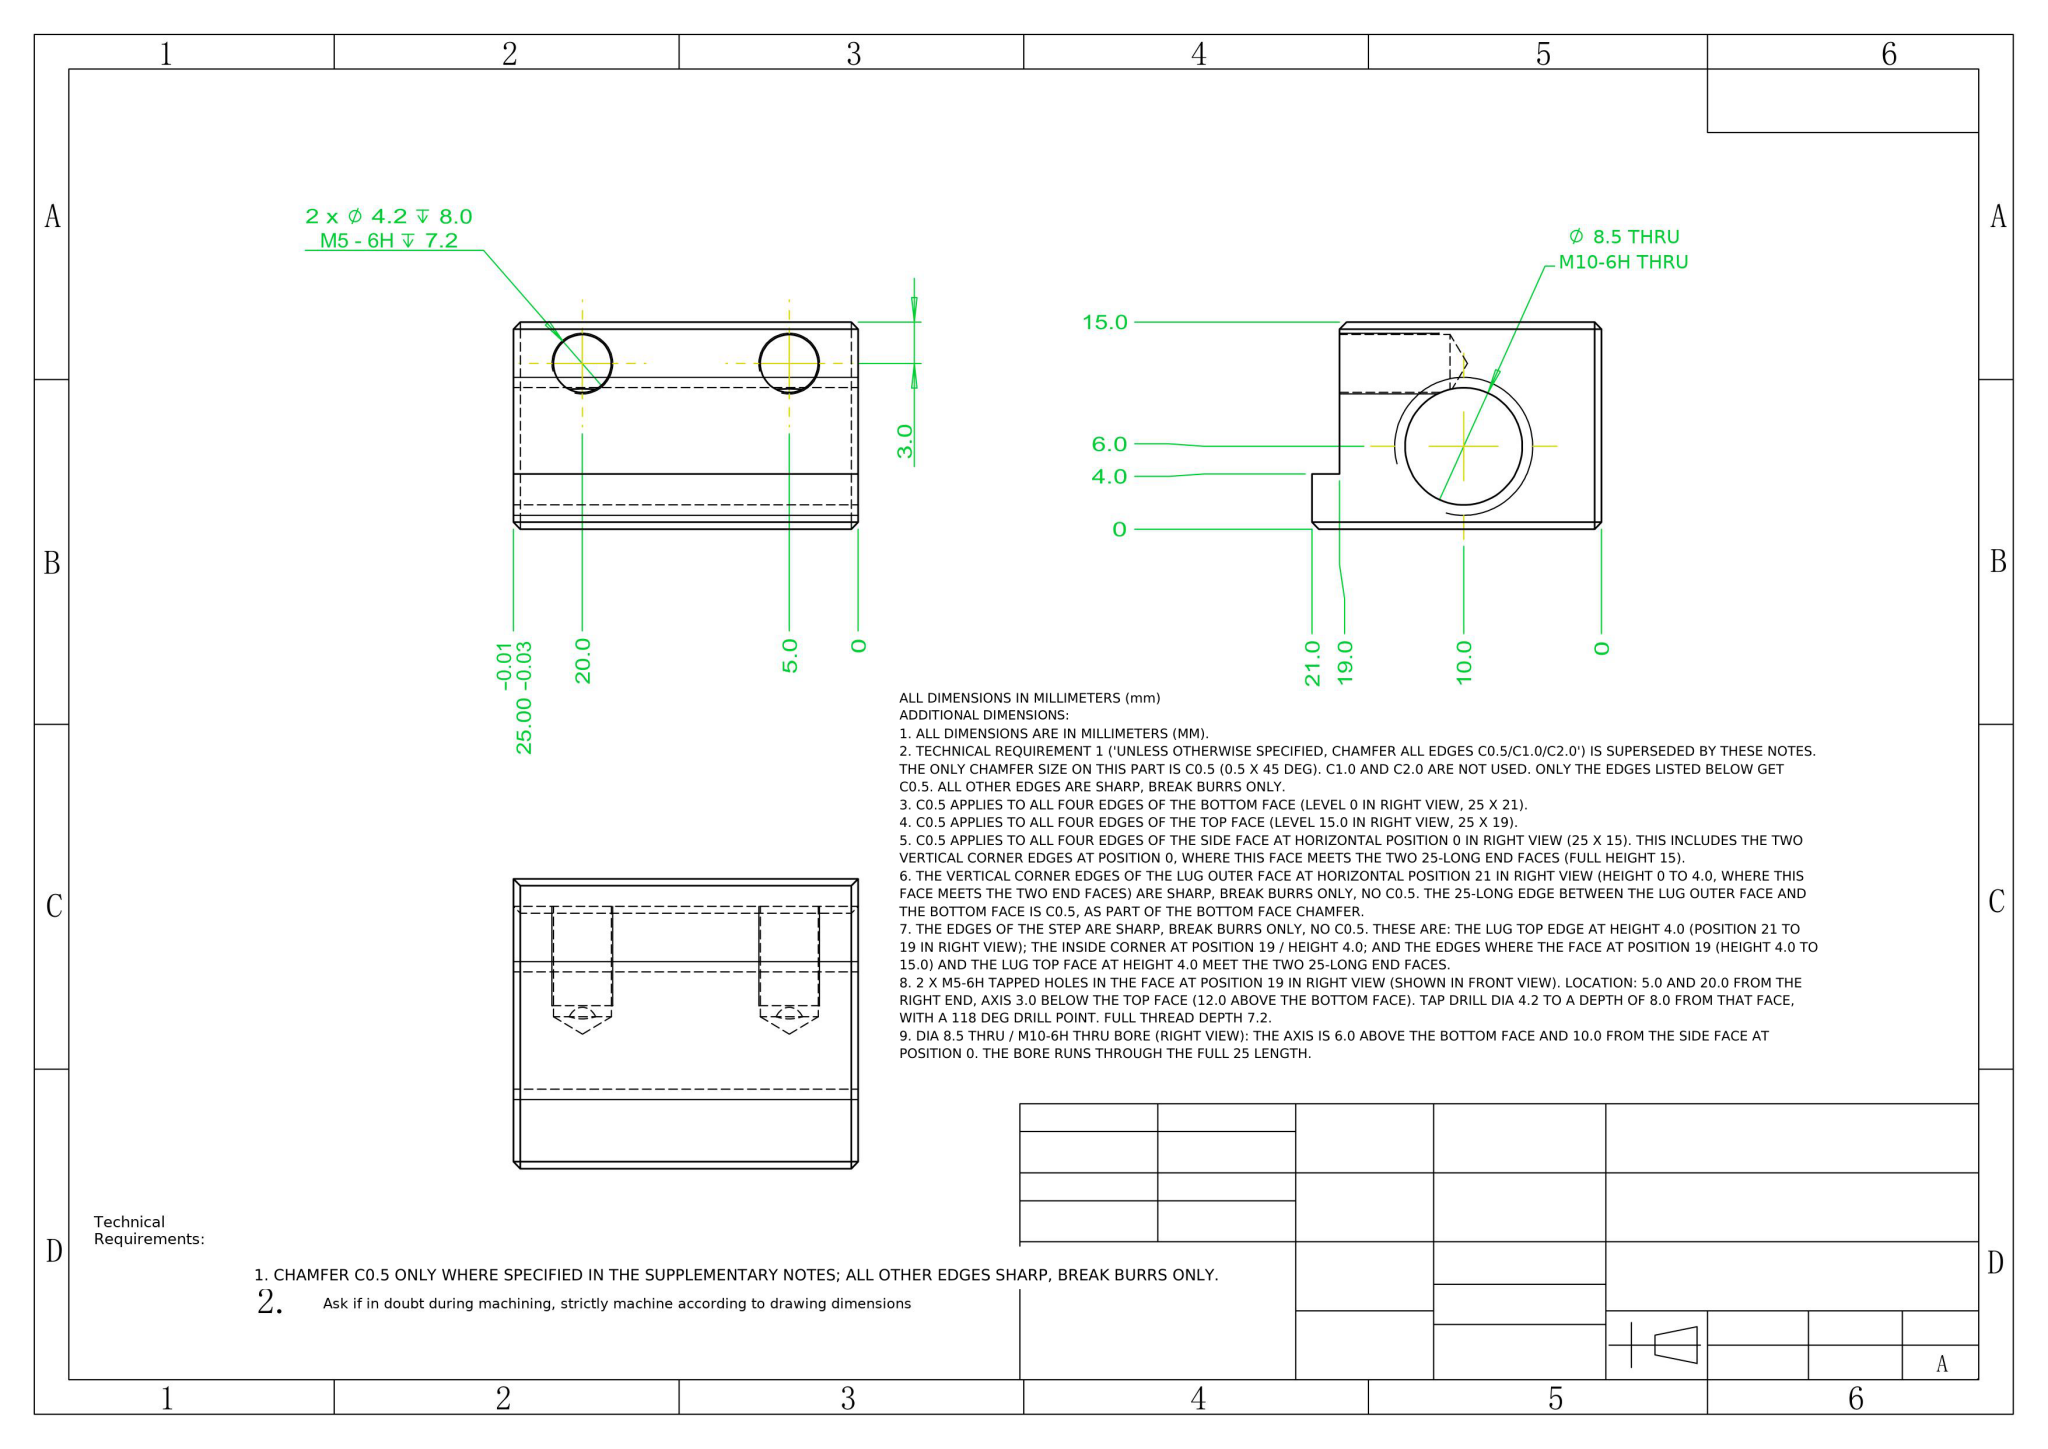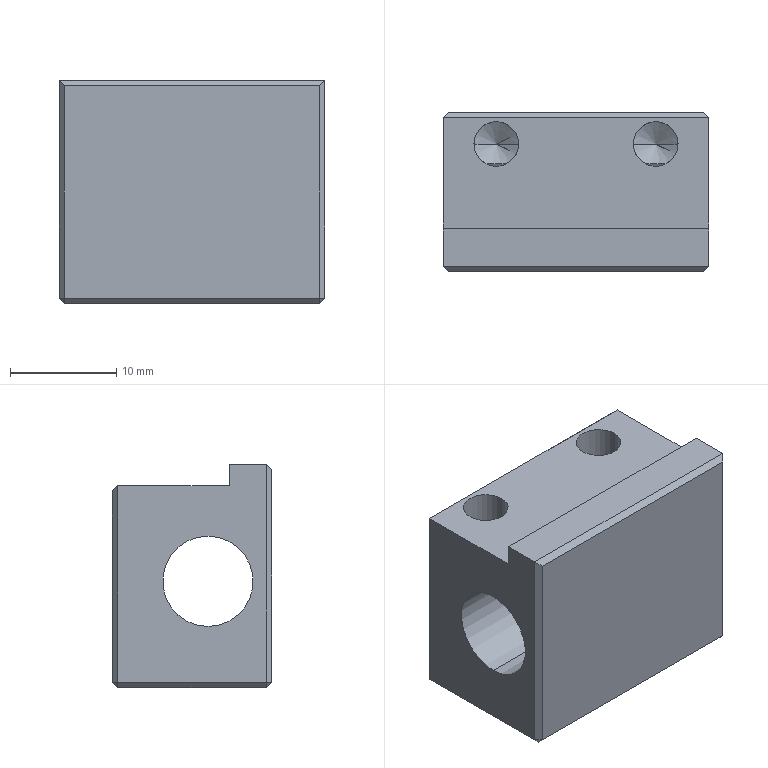Part | NX | mm | Tabbed Cylindrical Bore Block | 1 solid | 32 faces | box 25 x 15 x 21 mm | volume 5648 mm3 | plane 22 | cylinder 6 | cone 4 | commonest cylinder face diameters 4.2 x4 8.5 x2